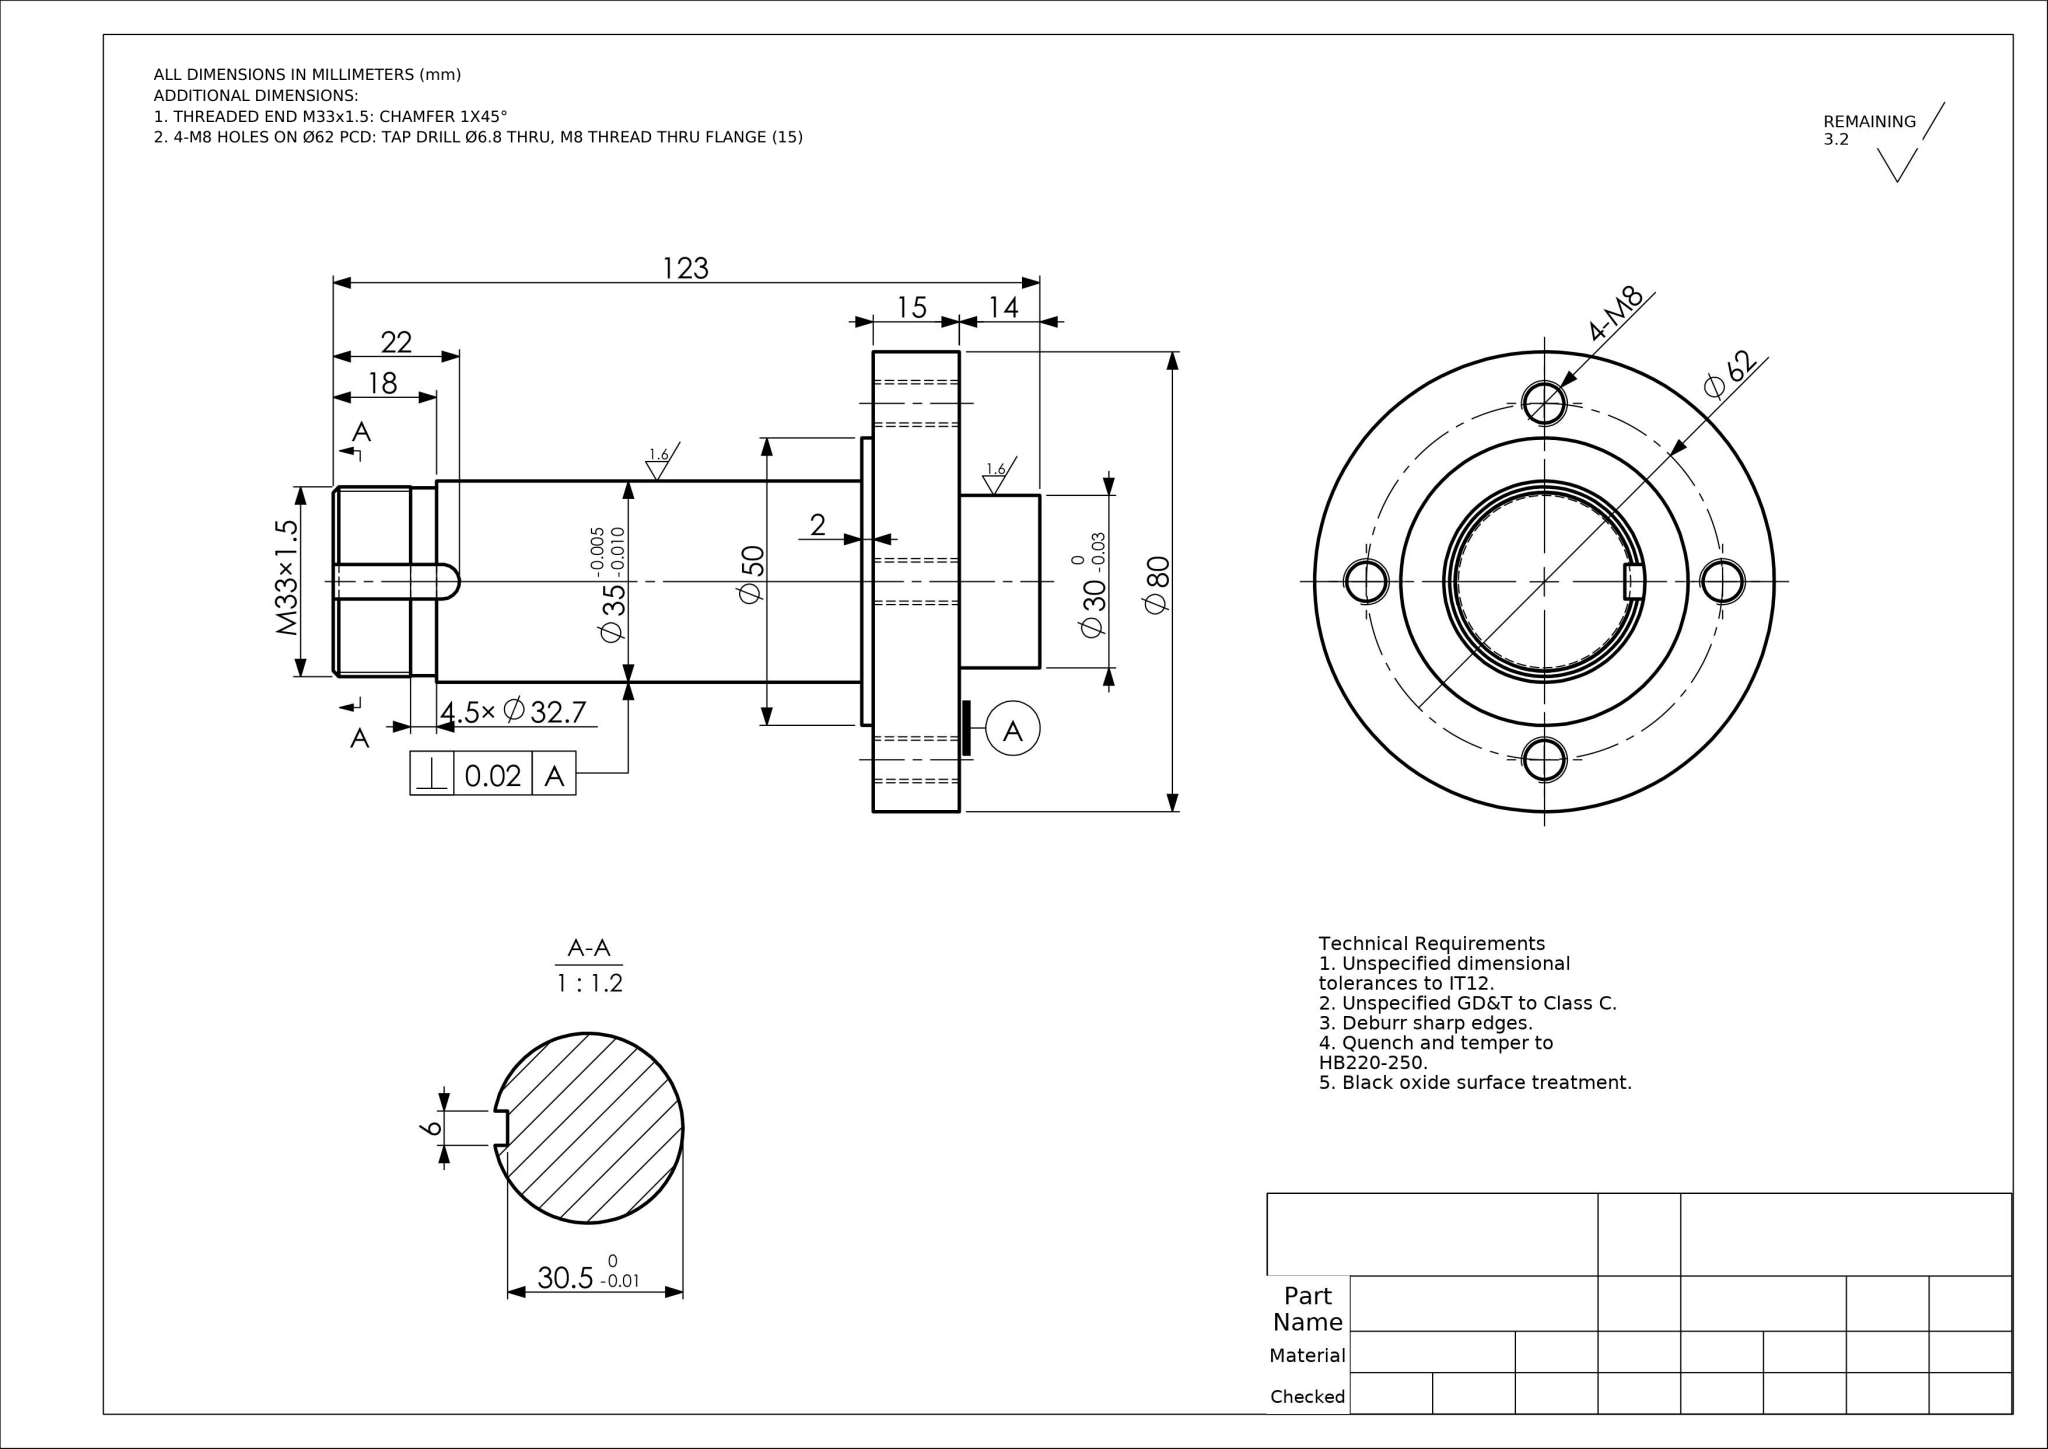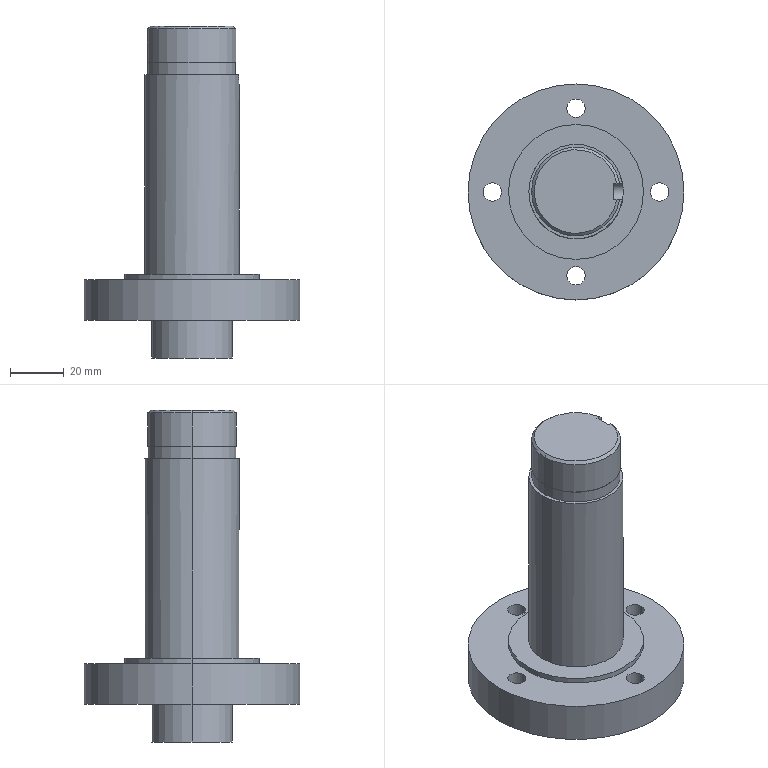Part | NX | mm | 1 solid | 33 faces | box 80 x 80 x 123 mm | volume 173191 mm3 | cylinder 21 | plane 10 | cone 2 | commonest cylinder face diameters 6.8 x8 50 x2 80 x2 30 x2 33 x2 32.7 x2 35 x2 6 x1